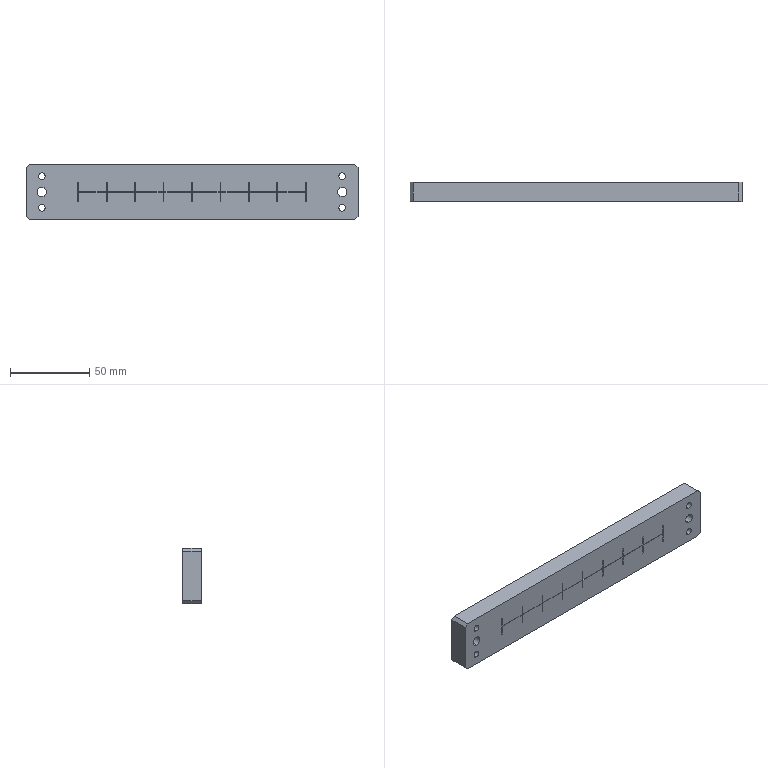Component | SolidWorks | 8TC-A15004-60-28A-2 | 1 solid | 90 faces | box 210 x 12 x 35 mm | volume 85766 mm3 | plane 78 | cylinder 12 | commonest cylinder face diameters 4.2 x8 6 x4 | material Cr12
build123d program:
from build123d import *

# Parameters (mm, degrees)
SKETCH1_W           = 210
SKETCH1_H           = 35
BOSS_EXTRUDE1_DEPTH = 6
SKETCH2_R           = 3
CUT_EXTRUDE1_DEPTH  = 20
CHAMFER1_SIZE       = 2
SKETCH6_W           = 0.5
SKETCH6_H           = 12.2
CUT_EXTRUDE3_DEPTH  = 108.123
LPATTERN1_COUNT     = 9
LPATTERN1_PITCH     = 18
M5_TAPPED_HOLE1_D   = 4.2
SKETCH9_W           = 144.13
SKETCH9_H           = 0.2
CUT_EXTRUDE4_DEPTH  = 108.123


with BuildPart() as part:
    # Sketch1 → Boss-Extrude1 (new, symmetric)
    with BuildSketch(Plane(origin=(0, 0, 0), x_dir=(1, 0, 0), z_dir=(0, 1, 0))):
        Rectangle(SKETCH1_W, SKETCH1_H)
    extrude(amount=BOSS_EXTRUDE1_DEPTH, both=True)

    # Sketch2 → Cut-Extrude1 (cut)
    with BuildSketch(Plane(origin=(0, 6, 0), x_dir=(1, 0, 0), z_dir=(0, 1, 0))):
        with Locations(Location((-95, 0, 0), (0, 0, 270))):
            Circle(SKETCH2_R)
        with Locations(Location((95, 0, 0), (0, 0, 90))):
            Circle(SKETCH2_R)
    extrude(amount=-CUT_EXTRUDE1_DEPTH, mode=Mode.SUBTRACT)

    # Chamfer1
    chamfer1_edges = [part.edges().sort_by_distance(p)[0] for p in [
        (105, 0, 17.5),
        (-105, 0, 17.5),
        (-105, 0, -17.5),
        (105, 0, -17.5),
    ]]
    chamfer(chamfer1_edges, length=CHAMFER1_SIZE)

    # Sketch6 → Cut-Extrude3 (cut, through all)
    with BuildSketch(Plane.XZ.offset(6)):
        with Locations((-72, 0)):
            Rectangle(SKETCH6_W, SKETCH6_H)
    cut_extrude3 = extrude(amount=-CUT_EXTRUDE3_DEPTH, mode=Mode.SUBTRACT)

    # LPattern1: Cut-Extrude3 ×9
    with Locations(*[(i * LPATTERN1_PITCH, 0, 0) for i in range(1, LPATTERN1_COUNT)]):
        add(cut_extrude3, mode=Mode.SUBTRACT)

    # M5 Tapped Hole1 (through all)
    with Locations(Plane(origin=(0, -6, 0), x_dir=(-1, 0, 0), z_dir=(0, -1, 0))):
        with Locations((95, 10), (95, -10), (-95, -10), (-95, 10)):
            Hole(M5_TAPPED_HOLE1_D / 2)

    # Sketch9 → Cut-Extrude4 (cut, through all)
    with BuildSketch(Plane.XZ.offset(6)):
        Rectangle(SKETCH9_W, SKETCH9_H)
    extrude(amount=-CUT_EXTRUDE4_DEPTH, mode=Mode.SUBTRACT)


solid = part.part

# Placed as in the assembly
solid = solid.moved(Location((26.714, -54, 0), (0, 0, 0)))